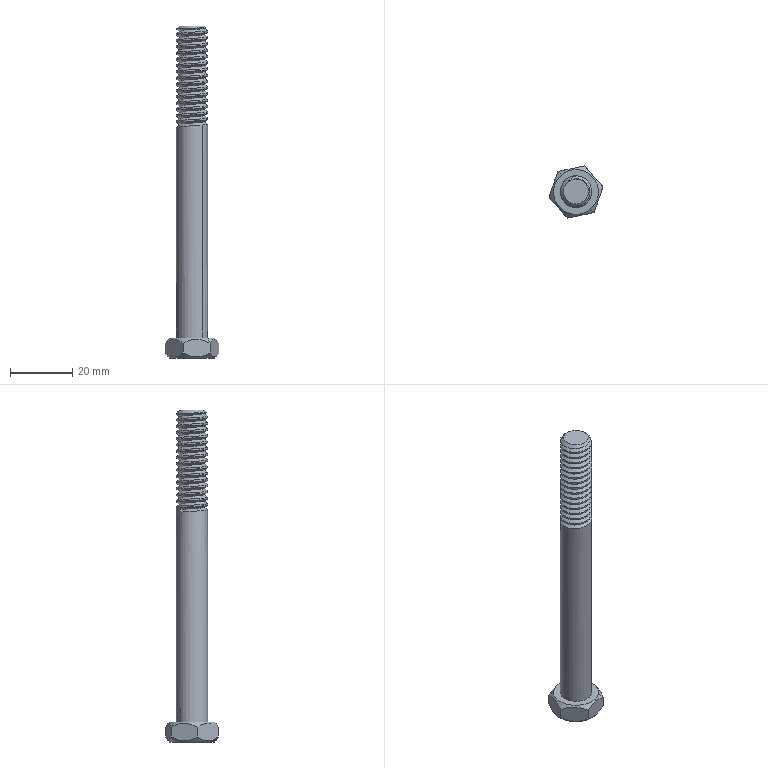Component | SolidWorks | M10-100-1 | 1 solid | 52 faces | volume 8741 mm3 | cylinder 33 | plane 10 | cone 7 | spline 2 | commonest cylinder face diameters 10 x33